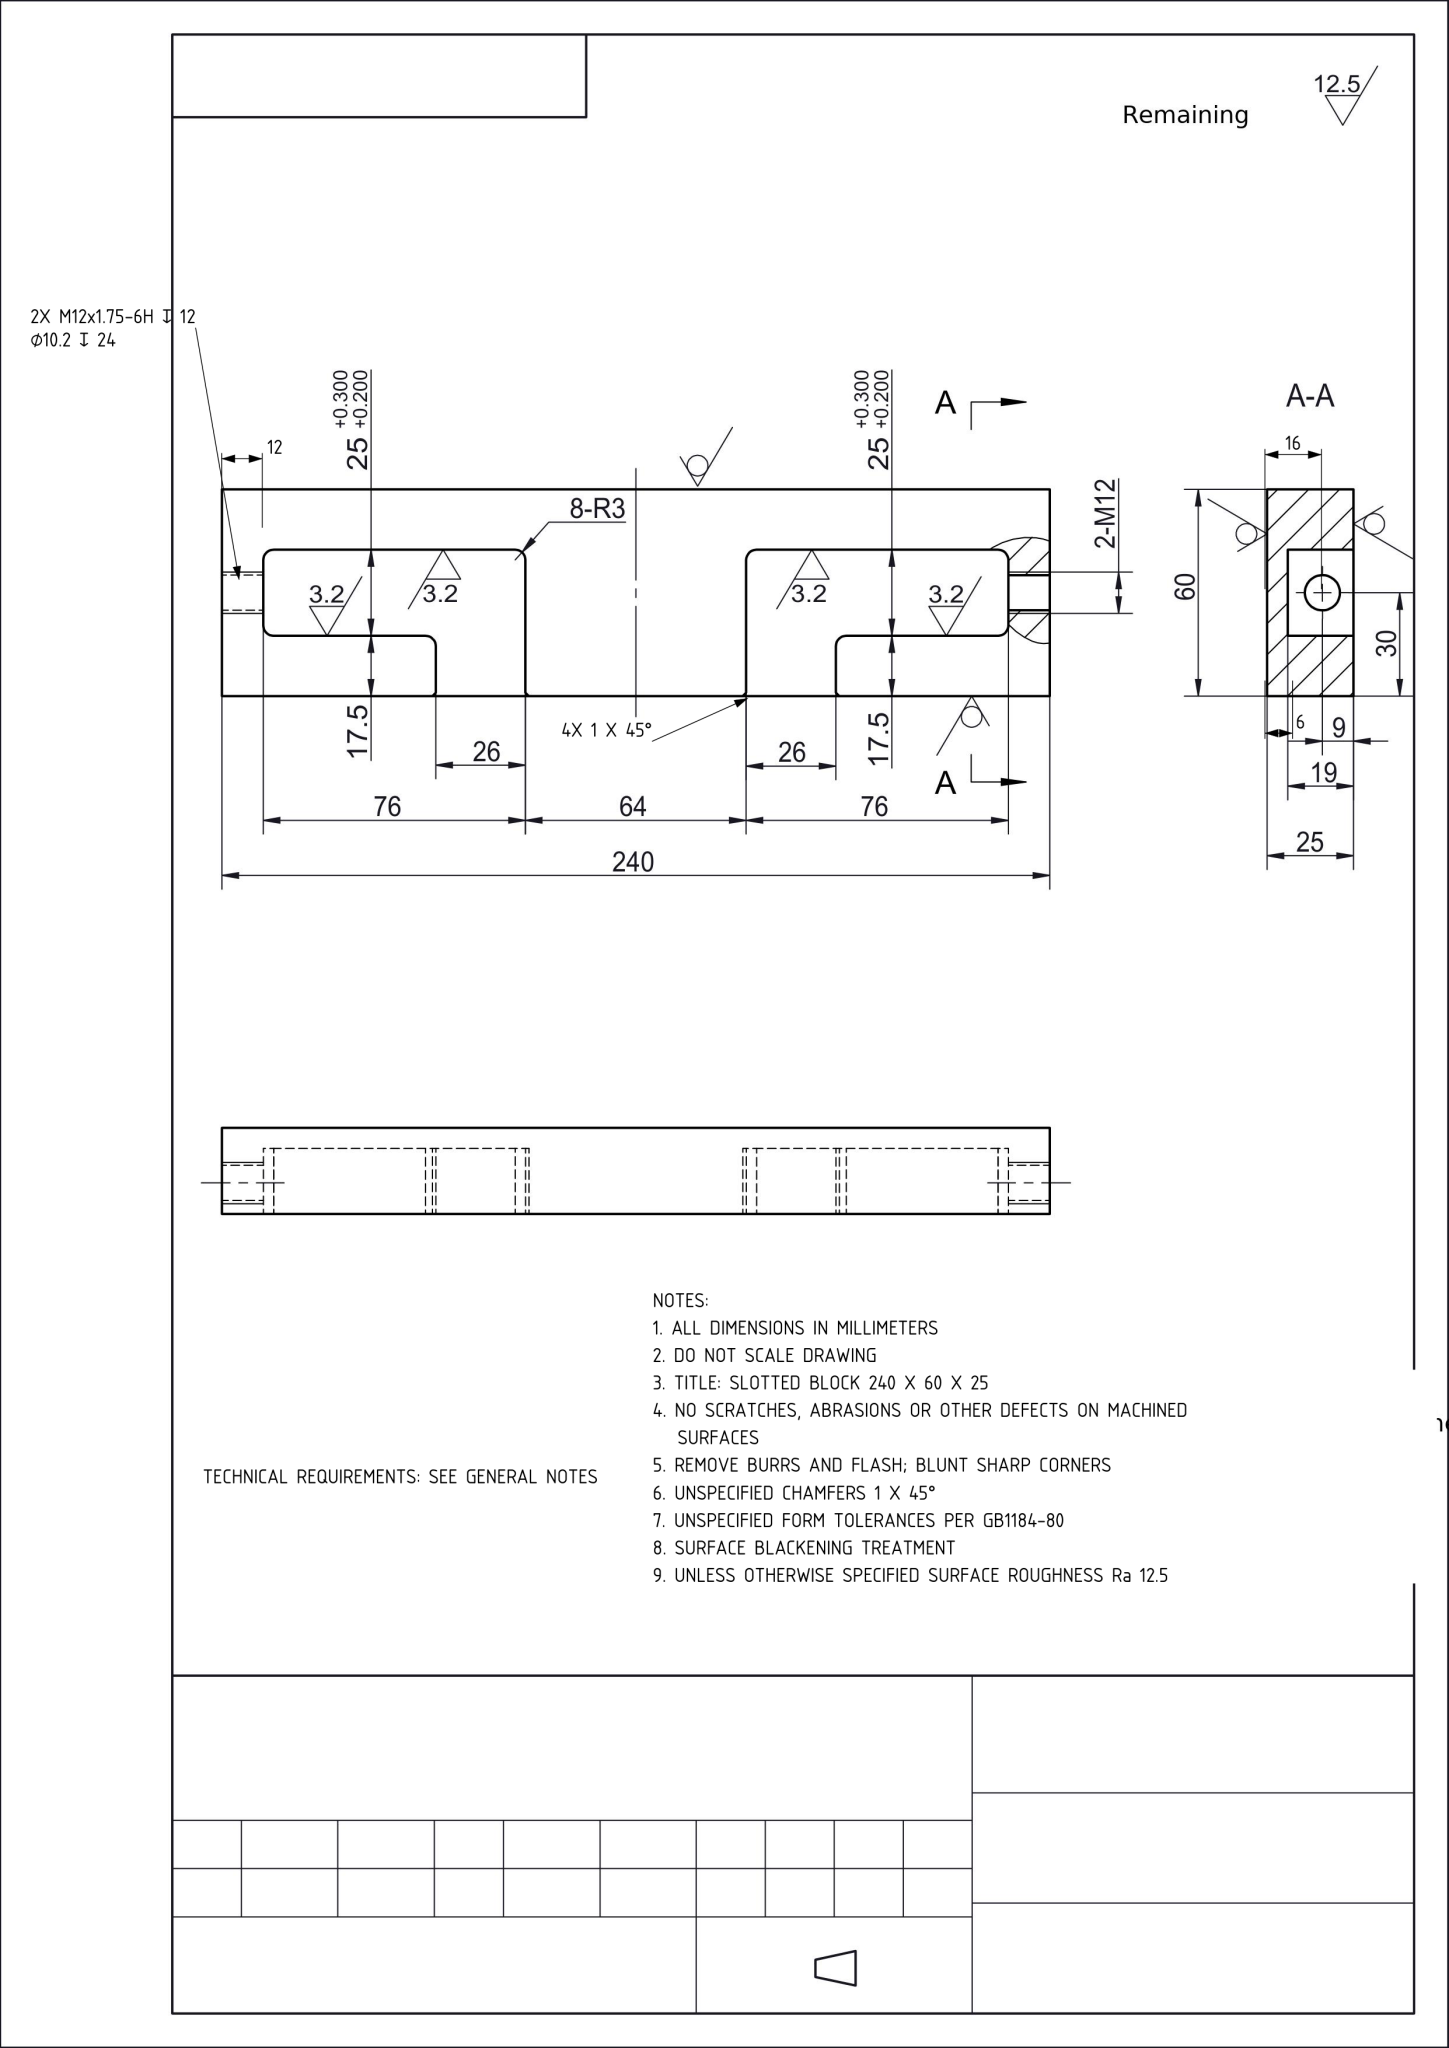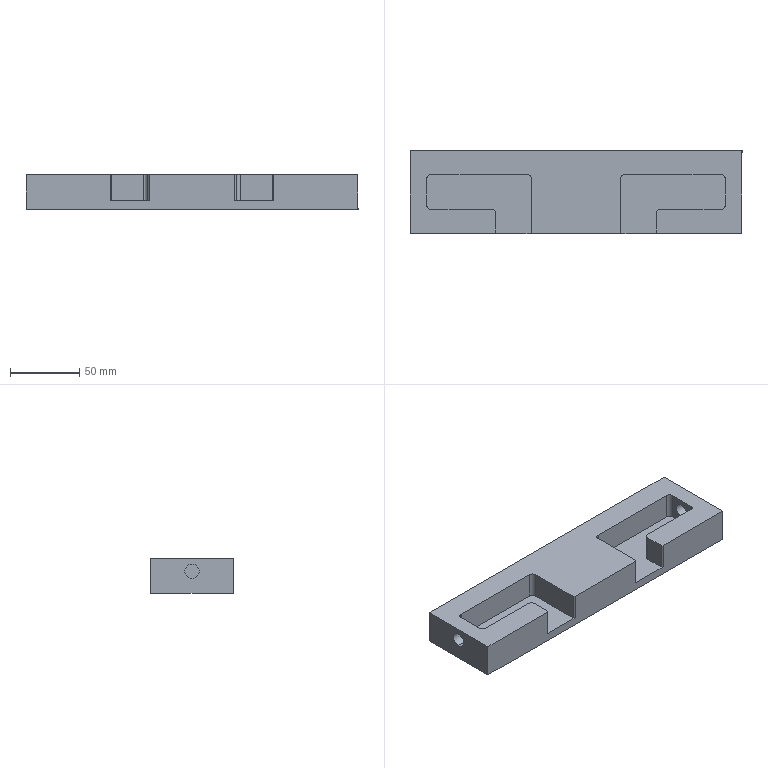Part | NX | mm | 1 solid | 34 faces | box 240 x 60 x 25 mm | volume 268658 mm3 | plane 22 | cylinder 12 | commonest cylinder face diameters 6 x8 10.2 x4